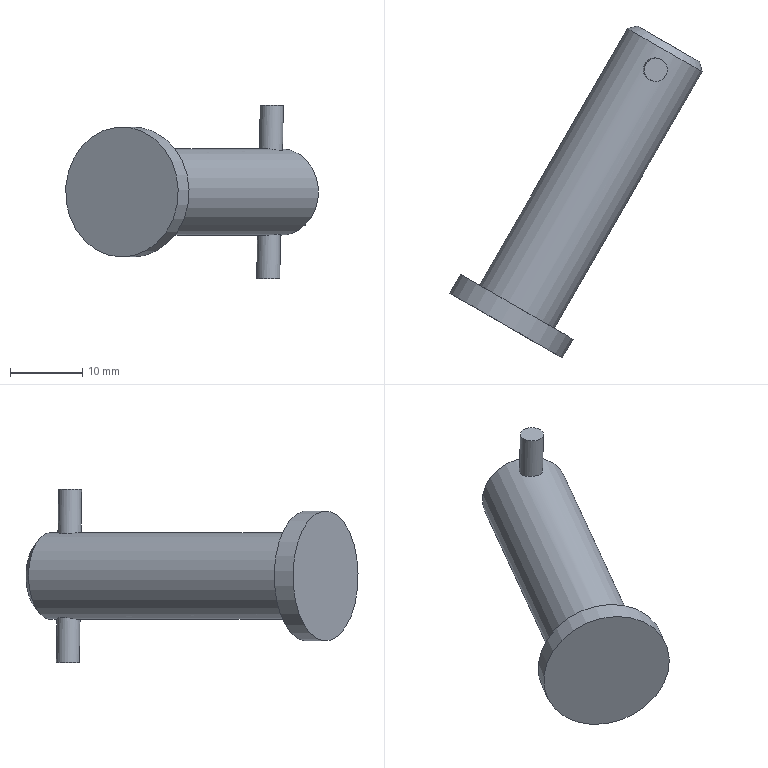Component | NX | PIN | 1 solid | 10 faces | volume 5593 mm3 | plane 5 | cylinder 4 | cone 1 | commonest cylinder face diameters 3.2 x2 12 x1 18 x1